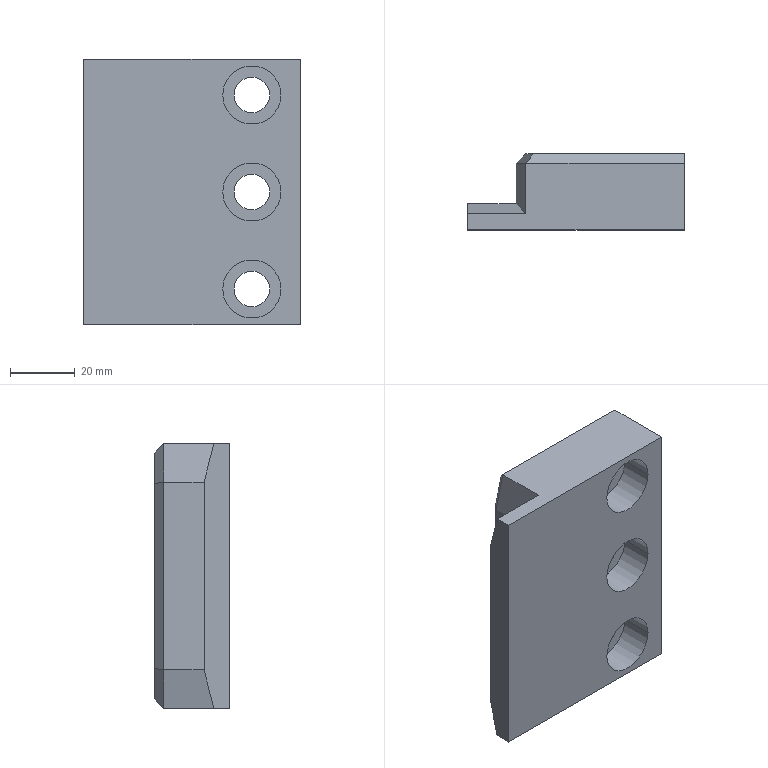Component | SolidWorks | EE8-213-_-_O-1 | 1 solid | 32 faces | box 67 x 23.5 x 82 mm | volume 96594 mm3 | plane 20 | cylinder 12 | commonest cylinder face diameters 18 x6 11 x6
build123d program:
from build123d import *
from OCP.BRepFilletAPI import BRepFilletAPI_MakeChamfer

# Parameters (mm, degrees)
EXTRUDE1_DEPTH                                       = 41
CHAMFER1_SIZE                                        = 3
CHAMFER1_SIZE2                                       = 12
CHAMFER2_SIZE                                        = 12
CHAMFER2_SIZE2                                       = 3
CHAMFER3_SIZE                                        = 3
COUNTERBORE_FOR_M10_SOCKET_HEAD_CAP_SCRE_D           = 11
COUNTERBORE_FOR_M10_SOCKET_HEAD_CAP_SCRE_CBORE_D     = 18
COUNTERBORE_FOR_M10_SOCKET_HEAD_CAP_SCRE_CBORE_DEPTH = 10


with BuildPart() as part:
    # Sketch1 → Extrude1 (new, symmetric)
    with BuildSketch(Plane(origin=(0, 0, 0), x_dir=(0, 0, -1), z_dir=(1, 0, 0))):
        Polygon((0, 0), (0, 23.5), (-52, 23.5), (-52, 8), (-67, 8), (-67, 0), align=None)
    extrude(amount=EXTRUDE1_DEPTH, both=True)

    # Chamfer1
    chamfer1_edges = [part.edges().sort_by_distance(p)[0] for p in [
        (-41, 8, 59.5),
        (-41, 15.75, 52),
    ]]
    chamfer1_side = [part.faces().sort_by_distance(p)[0] for p in [
        (-41, 11.057, 28.996),
    ]]
    chamfer(chamfer1_edges, length=CHAMFER1_SIZE, length2=CHAMFER1_SIZE2, reference=chamfer1_side[0])

    # Chamfer2: one chamfer whose edges measure the first distance from different faces: ONE call of the kernel's chamfer builder (chamfer() names one face for all edges)
    chamfer2_edges_1 = [part.edges().sort_by_distance(p)[0] for p in [
        (41, 15.75, 52),
    ]]
    chamfer2_side_1 = [part.faces().sort_by_distance(p)[0] for p in [
        (6, 15.75, 52),
    ]]
    chamfer2_edges_2 = [part.edges().sort_by_distance(p)[0] for p in [
        (41, 8, 59.5),
    ]]
    chamfer2_side_2 = [part.faces().sort_by_distance(p)[0] for p in [
        (6, 8, 59.5),
    ]]
    chamfer2 = BRepFilletAPI_MakeChamfer(part.part.solid().wrapped)
    for e in chamfer2_edges_1:
        chamfer2.Add(CHAMFER2_SIZE, CHAMFER2_SIZE2, e.wrapped, chamfer2_side_1[0].wrapped)  # the first distance lies on this face
    for e in chamfer2_edges_2:
        chamfer2.Add(CHAMFER2_SIZE, CHAMFER2_SIZE2, e.wrapped, chamfer2_side_2[0].wrapped)  # the first distance lies on this face
    add(Compound.cast(chamfer2.Shape()), mode=Mode.REPLACE)

    # Chamfer3
    chamfer3_edges = [part.edges().sort_by_distance(p)[0] for p in [
        (41, 23.5, 24.5),
        (-35, 23.5, 50.5),
        (0, 23.5, 52),
        (35, 23.5, 50.5),
        (-41, 23.5, 24.5),
    ]]
    chamfer(chamfer3_edges, length=CHAMFER3_SIZE)

    # Counterbore for M10 Socket Head Cap Scre (through all)
    with Locations(Plane.XZ):
        with Locations((0, 15), (-30, 15), (30, 15)):
            CounterBoreHole(COUNTERBORE_FOR_M10_SOCKET_HEAD_CAP_SCRE_D / 2, COUNTERBORE_FOR_M10_SOCKET_HEAD_CAP_SCRE_CBORE_D / 2, COUNTERBORE_FOR_M10_SOCKET_HEAD_CAP_SCRE_CBORE_DEPTH)


solid = part.part

# Placed as in the assembly
solid = solid.moved(Location((15, -23.5, 245), (0, -90, 0)))
STEP:
#1=CARTESIAN_POINT('',(-0.3543,-0.5315,8.465));
#2=VERTEX_POINT('',#1);
#3=CARTESIAN_POINT('',(0.3543,-0.5315,8.465));
#4=VERTEX_POINT('',#3);
#5=CARTESIAN_POINT('',(0.,-0.5315,8.465));
#6=DIRECTION('',(0.,-1.,0.));
#7=DIRECTION('',(1.,0.,-0.));
#8=AXIS2_PLACEMENT_3D('',#5,#6,#7);
#9=CIRCLE('',#8,0.3543);
#10=EDGE_CURVE('',#2,#4,#9,.T.);
#11=ORIENTED_EDGE('',*,*,#10,.F.);
#12=CARTESIAN_POINT('',(-0.3543,-0.9252,8.465));
#13=VERTEX_POINT('',#12);
#14=CARTESIAN_POINT('',(-0.3543,-0.9252,8.465));
#15=DIRECTION('',(0.,-1.,0.));
#16=VECTOR('',#15,39.37);
#17=LINE('',#14,#16);
#18=EDGE_CURVE('',#2,#13,#17,.T.);
#19=ORIENTED_EDGE('',*,*,#18,.T.);
#20=CARTESIAN_POINT('',(0.3543,-0.9252,8.465));
#21=VERTEX_POINT('',#20);
#22=CARTESIAN_POINT('',(0.,-0.9252,8.465));
#23=DIRECTION('',(0.,-1.,0.));
#24=DIRECTION('',(1.,0.,-0.));
#25=AXIS2_PLACEMENT_3D('',#22,#23,#24);
#26=CIRCLE('',#25,0.3543);
#27=EDGE_CURVE('',#13,#21,#26,.T.);
#28=ORIENTED_EDGE('',*,*,#27,.T.);
#29=CARTESIAN_POINT('',(0.3543,-0.9252,8.465));
#30=DIRECTION('',(0.,-1.,0.));
#31=VECTOR('',#30,39.37);
#32=LINE('',#29,#31);
#33=EDGE_CURVE('',#4,#21,#32,.T.);
#34=ORIENTED_EDGE('',*,*,#33,.F.);
#35=EDGE_LOOP('',(#11,#19,#28,#34));
#36=FACE_OUTER_BOUND('',#35,.T.);
#37=CARTESIAN_POINT('',(0.,-0.9252,8.465));
#38=DIRECTION('',(0.,-1.,0.));
#39=DIRECTION('',(1.,0.,-0.));
#40=AXIS2_PLACEMENT_3D('',#37,#38,#39);
#41=CYLINDRICAL_SURFACE('',#40,0.3543);
#42=ADVANCED_FACE('',(#36),#41,.F.);
#43=CARTESIAN_POINT('',(-0.2165,0.,8.465));
#44=VERTEX_POINT('',#43);
#45=CARTESIAN_POINT('',(0.2165,0.,8.465));
#46=VERTEX_POINT('',#45);
#47=CARTESIAN_POINT('',(0.,0.,8.465));
#48=DIRECTION('',(0.,-1.,0.));
#49=DIRECTION('',(1.,0.,-0.));
#50=AXIS2_PLACEMENT_3D('',#47,#48,#49);
#51=CIRCLE('',#50,0.2165);
#52=EDGE_CURVE('',#44,#46,#51,.T.);
#53=ORIENTED_EDGE('',*,*,#52,.F.);
#54=CARTESIAN_POINT('',(-0.2165,-0.5315,8.465));
#55=VERTEX_POINT('',#54);
#56=CARTESIAN_POINT('',(-0.2165,-0.9252,8.465));
#57=DIRECTION('',(0.,-1.,0.));
#58=VECTOR('',#57,39.37);
#59=LINE('',#56,#58);
#60=EDGE_CURVE('',#44,#55,#59,.T.);
#61=ORIENTED_EDGE('',*,*,#60,.T.);
#62=CARTESIAN_POINT('',(0.2165,-0.5315,8.465));
#63=VERTEX_POINT('',#62);
#64=CARTESIAN_POINT('',(0.,-0.5315,8.465));
#65=DIRECTION('',(0.,-1.,0.));
#66=DIRECTION('',(1.,0.,-0.));
#67=AXIS2_PLACEMENT_3D('',#64,#65,#66);
#68=CIRCLE('',#67,0.2165);
#69=EDGE_CURVE('',#55,#63,#68,.T.);
#70=ORIENTED_EDGE('',*,*,#69,.T.);
#71=CARTESIAN_POINT('',(0.2165,-0.9252,8.465));
#72=DIRECTION('',(0.,-1.,0.));
#73=VECTOR('',#72,39.37);
#74=LINE('',#71,#73);
#75=EDGE_CURVE('',#46,#63,#74,.T.);
#76=ORIENTED_EDGE('',*,*,#75,.F.);
#77=EDGE_LOOP('',(#53,#61,#70,#76));
#78=FACE_OUTER_BOUND('',#77,.T.);
#79=CARTESIAN_POINT('',(0.,-0.9252,8.465));
#80=DIRECTION('',(0.,-1.,0.));
#81=DIRECTION('',(1.,0.,-0.));
#82=AXIS2_PLACEMENT_3D('',#79,#80,#81);
#83=CYLINDRICAL_SURFACE('',#82,0.2165);
#84=ADVANCED_FACE('',(#78),#83,.F.);
#85=CARTESIAN_POINT('',(-0.3543,-0.5315,10.827));
#86=VERTEX_POINT('',#85);
#87=CARTESIAN_POINT('',(0.3543,-0.5315,10.827));
#88=VERTEX_POINT('',#87);
#89=CARTESIAN_POINT('',(0.,-0.5315,10.827));
#90=DIRECTION('',(0.,-1.,0.));
#91=DIRECTION('',(1.,0.,-0.));
#92=AXIS2_PLACEMENT_3D('',#89,#90,#91);
#93=CIRCLE('',#92,0.3543);
#94=EDGE_CURVE('',#86,#88,#93,.T.);
#95=ORIENTED_EDGE('',*,*,#94,.F.);
#96=CARTESIAN_POINT('',(-0.3543,-0.9252,10.827));
#97=VERTEX_POINT('',#96);
#98=CARTESIAN_POINT('',(-0.3543,-0.9252,10.827));
#99=DIRECTION('',(0.,-1.,0.));
#100=VECTOR('',#99,39.37);
#101=LINE('',#98,#100);
#102=EDGE_CURVE('',#86,#97,#101,.T.);
#103=ORIENTED_EDGE('',*,*,#102,.T.);
#104=CARTESIAN_POINT('',(0.3543,-0.9252,10.827));
#105=VERTEX_POINT('',#104);
#106=CARTESIAN_POINT('',(0.,-0.9252,10.827));
#107=DIRECTION('',(0.,-1.,0.));
#108=DIRECTION('',(1.,0.,-0.));
#109=AXIS2_PLACEMENT_3D('',#106,#107,#108);
#110=CIRCLE('',#109,0.3543);
#111=EDGE_CURVE('',#97,#105,#110,.T.);
#112=ORIENTED_EDGE('',*,*,#111,.T.);
#113=CARTESIAN_POINT('',(0.3543,-0.9252,10.827));
#114=DIRECTION('',(0.,-1.,0.));
#115=VECTOR('',#114,39.37);
#116=LINE('',#113,#115);
#117=EDGE_CURVE('',#88,#105,#116,.T.);
#118=ORIENTED_EDGE('',*,*,#117,.F.);
#119=EDGE_LOOP('',(#95,#103,#112,#118));
#120=FACE_OUTER_BOUND('',#119,.T.);
#121=CARTESIAN_POINT('',(0.,-0.9252,10.827));
#122=DIRECTION('',(0.,-1.,0.));
#123=DIRECTION('',(1.,0.,-0.));
#124=AXIS2_PLACEMENT_3D('',#121,#122,#123);
#125=CYLINDRICAL_SURFACE('',#124,0.3543);
#126=ADVANCED_FACE('',(#120),#125,.F.);
#127=CARTESIAN_POINT('',(-0.2165,0.,10.827));
#128=VERTEX_POINT('',#127);
#129=CARTESIAN_POINT('',(0.2165,0.,10.827));
#130=VERTEX_POINT('',#129);
#131=CARTESIAN_POINT('',(0.,0.,10.827));
#132=DIRECTION('',(0.,-1.,0.));
#133=DIRECTION('',(1.,0.,0.));
#134=AXIS2_PLACEMENT_3D('',#131,#132,#133);
#135=CIRCLE('',#134,0.2165);
#136=EDGE_CURVE('',#128,#130,#135,.T.);
#137=ORIENTED_EDGE('',*,*,#136,.F.);
#138=CARTESIAN_POINT('',(-0.2165,-0.5315,10.827));
#139=VERTEX_POINT('',#138);
#140=CARTESIAN_POINT('',(-0.2165,-0.9252,10.827));
#141=DIRECTION('',(0.,-1.,0.));
#142=VECTOR('',#141,39.37);
#143=LINE('',#140,#142);
#144=EDGE_CURVE('',#128,#139,#143,.T.);
#145=ORIENTED_EDGE('',*,*,#144,.T.);
#146=CARTESIAN_POINT('',(0.2165,-0.5315,10.827));
#147=VERTEX_POINT('',#146);
#148=CARTESIAN_POINT('',(0.,-0.5315,10.827));
#149=DIRECTION('',(0.,-1.,0.));
#150=DIRECTION('',(1.,0.,0.));
#151=AXIS2_PLACEMENT_3D('',#148,#149,#150);
#152=CIRCLE('',#151,0.2165);
#153=EDGE_CURVE('',#139,#147,#152,.T.);
#154=ORIENTED_EDGE('',*,*,#153,.T.);
#155=CARTESIAN_POINT('',(0.2165,-0.9252,10.827));
#156=DIRECTION('',(0.,-1.,0.));
#157=VECTOR('',#156,39.37);
#158=LINE('',#155,#157);
#159=EDGE_CURVE('',#130,#147,#158,.T.);
#160=ORIENTED_EDGE('',*,*,#159,.F.);
#161=EDGE_LOOP('',(#137,#145,#154,#160));
#162=FACE_OUTER_BOUND('',#161,.T.);
#163=CARTESIAN_POINT('',(0.,-0.9252,10.827));
#164=DIRECTION('',(0.,-1.,0.));
#165=DIRECTION('',(1.,0.,0.));
#166=AXIS2_PLACEMENT_3D('',#163,#164,#165);
#167=CYLINDRICAL_SURFACE('',#166,0.2165);
#168=ADVANCED_FACE('',(#162),#167,.F.);
#169=CARTESIAN_POINT('',(-0.3543,-0.5315,9.646));
#170=VERTEX_POINT('',#169);
#171=CARTESIAN_POINT('',(0.3543,-0.5315,9.646));
#172=VERTEX_POINT('',#171);
#173=CARTESIAN_POINT('',(0.,-0.5315,9.646));
#174=DIRECTION('',(0.,-1.,0.));
#175=DIRECTION('',(1.,0.,-0.));
#176=AXIS2_PLACEMENT_3D('',#173,#174,#175);
#177=CIRCLE('',#176,0.3543);
#178=EDGE_CURVE('',#170,#172,#177,.T.);
#179=ORIENTED_EDGE('',*,*,#178,.F.);
#180=CARTESIAN_POINT('',(-0.3543,-0.9252,9.646));
#181=VERTEX_POINT('',#180);
#182=CARTESIAN_POINT('',(-0.3543,-0.9252,9.646));
#183=DIRECTION('',(0.,-1.,0.));
#184=VECTOR('',#183,39.37);
#185=LINE('',#182,#184);
#186=EDGE_CURVE('',#170,#181,#185,.T.);
#187=ORIENTED_EDGE('',*,*,#186,.T.);
#188=CARTESIAN_POINT('',(0.3543,-0.9252,9.646));
#189=VERTEX_POINT('',#188);
#190=CARTESIAN_POINT('',(0.,-0.9252,9.646));
#191=DIRECTION('',(0.,-1.,0.));
#192=DIRECTION('',(1.,0.,-0.));
#193=AXIS2_PLACEMENT_3D('',#190,#191,#192);
#194=CIRCLE('',#193,0.3543);
#195=EDGE_CURVE('',#181,#189,#194,.T.);
#196=ORIENTED_EDGE('',*,*,#195,.T.);
#197=CARTESIAN_POINT('',(0.3543,-0.9252,9.646));
#198=DIRECTION('',(0.,-1.,0.));
#199=VECTOR('',#198,39.37);
#200=LINE('',#197,#199);
#201=EDGE_CURVE('',#172,#189,#200,.T.);
#202=ORIENTED_EDGE('',*,*,#201,.F.);
#203=EDGE_LOOP('',(#179,#187,#196,#202));
#204=FACE_OUTER_BOUND('',#203,.T.);
#205=CARTESIAN_POINT('',(0.,-0.9252,9.646));
#206=DIRECTION('',(0.,-1.,0.));
#207=DIRECTION('',(1.,0.,-0.));
#208=AXIS2_PLACEMENT_3D('',#205,#206,#207);
#209=CYLINDRICAL_SURFACE('',#208,0.3543);
#210=ADVANCED_FACE('',(#204),#209,.F.);
#211=CARTESIAN_POINT('',(-0.2165,0.,9.646));
#212=VERTEX_POINT('',#211);
#213=CARTESIAN_POINT('',(0.2165,0.,9.646));
#214=VERTEX_POINT('',#213);
#215=CARTESIAN_POINT('',(0.,0.,9.646));
#216=DIRECTION('',(0.,-1.,0.));
#217=DIRECTION('',(1.,0.,-0.));
#218=AXIS2_PLACEMENT_3D('',#215,#216,#217);
#219=CIRCLE('',#218,0.2165);
#220=EDGE_CURVE('',#212,#214,#219,.T.);
#221=ORIENTED_EDGE('',*,*,#220,.F.);
#222=CARTESIAN_POINT('',(-0.2165,-0.5315,9.646));
#223=VERTEX_POINT('',#222);
#224=CARTESIAN_POINT('',(-0.2165,-0.9252,9.646));
#225=DIRECTION('',(0.,-1.,0.));
#226=VECTOR('',#225,39.37);
#227=LINE('',#224,#226);
#228=EDGE_CURVE('',#212,#223,#227,.T.);
#229=ORIENTED_EDGE('',*,*,#228,.T.);
#230=CARTESIAN_POINT('',(0.2165,-0.5315,9.646));
#231=VERTEX_POINT('',#230);
#232=CARTESIAN_POINT('',(0.,-0.5315,9.646));
#233=DIRECTION('',(0.,-1.,0.));
#234=DIRECTION('',(1.,0.,-0.));
#235=AXIS2_PLACEMENT_3D('',#232,#233,#234);
#236=CIRCLE('',#235,0.2165);
#237=EDGE_CURVE('',#223,#231,#236,.T.);
#238=ORIENTED_EDGE('',*,*,#237,.T.);
#239=CARTESIAN_POINT('',(0.2165,-0.9252,9.646));
#240=DIRECTION('',(0.,-1.,0.));
#241=VECTOR('',#240,39.37);
#242=LINE('',#239,#241);
#243=EDGE_CURVE('',#214,#231,#242,.T.);
#244=ORIENTED_EDGE('',*,*,#243,.F.);
#245=EDGE_LOOP('',(#221,#229,#238,#244));
#246=FACE_OUTER_BOUND('',#245,.T.);
#247=CARTESIAN_POINT('',(0.,-0.9252,9.646));
#248=DIRECTION('',(0.,-1.,0.));
#249=DIRECTION('',(1.,0.,-0.));
#250=AXIS2_PLACEMENT_3D('',#247,#248,#249);
#251=CYLINDRICAL_SURFACE('',#250,0.2165);
#252=ADVANCED_FACE('',(#246),#251,.F.);
#253=CARTESIAN_POINT('',(0.,-0.9252,8.465));
#254=DIRECTION('',(0.,-1.,0.));
#255=DIRECTION('',(1.,0.,-0.));
#256=AXIS2_PLACEMENT_3D('',#253,#254,#255);
#257=CIRCLE('',#256,0.3543);
#258=EDGE_CURVE('',#21,#13,#257,.T.);
#259=ORIENTED_EDGE('',*,*,#258,.F.);
#260=ORIENTED_EDGE('',*,*,#27,.F.);
#261=EDGE_LOOP('',(#259,#260));
#262=FACE_BOUND('',#261,.T.);
#263=CARTESIAN_POINT('',(0.,-0.9252,10.827));
#264=DIRECTION('',(0.,-1.,0.));
#265=DIRECTION('',(1.,0.,-0.));
#266=AXIS2_PLACEMENT_3D('',#263,#264,#265);
#267=CIRCLE('',#266,0.3543);
#268=EDGE_CURVE('',#105,#97,#267,.T.);
#269=ORIENTED_EDGE('',*,*,#268,.F.);
#270=ORIENTED_EDGE('',*,*,#111,.F.);
#271=EDGE_LOOP('',(#269,#270));
#272=FACE_BOUND('',#271,.T.);
#273=CARTESIAN_POINT('',(0.,-0.9252,9.646));
#274=DIRECTION('',(0.,-1.,0.));
#275=DIRECTION('',(1.,0.,-0.));
#276=AXIS2_PLACEMENT_3D('',#273,#274,#275);
#277=CIRCLE('',#276,0.3543);
#278=EDGE_CURVE('',#189,#181,#277,.T.);
#279=ORIENTED_EDGE('',*,*,#278,.F.);
#280=ORIENTED_EDGE('',*,*,#195,.F.);
#281=EDGE_LOOP('',(#279,#280));
#282=FACE_BOUND('',#281,.T.);
#283=CARTESIAN_POINT('',(-2.047,-0.9252,8.031));
#284=VERTEX_POINT('',#283);
#285=CARTESIAN_POINT('',(0.5906,-0.9252,8.031));
#286=VERTEX_POINT('',#285);
#287=CARTESIAN_POINT('',(-2.047,-0.9252,8.031));
#288=DIRECTION('',(1.,0.,-0.));
#289=VECTOR('',#288,39.37);
#290=LINE('',#287,#289);
#291=EDGE_CURVE('',#284,#286,#290,.T.);
#292=ORIENTED_EDGE('',*,*,#291,.T.);
#293=CARTESIAN_POINT('',(0.5906,-0.9252,11.26));
#294=VERTEX_POINT('',#293);
#295=CARTESIAN_POINT('',(0.5906,-0.9252,11.26));
#296=DIRECTION('',(-0.,0.,-1.));
#297=VECTOR('',#296,39.37);
#298=LINE('',#295,#297);
#299=EDGE_CURVE('',#294,#286,#298,.T.);
#300=ORIENTED_EDGE('',*,*,#299,.F.);
#301=CARTESIAN_POINT('',(-2.047,-0.9252,11.26));
#302=VERTEX_POINT('',#301);
#303=CARTESIAN_POINT('',(-2.047,-0.9252,11.26));
#304=DIRECTION('',(1.,0.,-0.));
#305=VECTOR('',#304,39.37);
#306=LINE('',#303,#305);
#307=EDGE_CURVE('',#302,#294,#306,.T.);
#308=ORIENTED_EDGE('',*,*,#307,.F.);
#309=CARTESIAN_POINT('',(-2.047,-0.9252,11.26));
#310=DIRECTION('',(-0.,0.,-1.));
#311=VECTOR('',#310,39.37);
#312=LINE('',#309,#311);
#313=EDGE_CURVE('',#302,#284,#312,.T.);
#314=ORIENTED_EDGE('',*,*,#313,.T.);
#315=EDGE_LOOP('',(#292,#300,#308,#314));
#316=FACE_OUTER_BOUND('',#315,.T.);
#317=CARTESIAN_POINT('',(-2.047,-0.9252,11.26));
#318=DIRECTION('',(0.,1.,0.));
#319=DIRECTION('',(-1.,0.,0.));
#320=AXIS2_PLACEMENT_3D('',#317,#318,#319);
#321=PLANE('',#320);
#322=ADVANCED_FACE('',(#262,#272,#282,#316),#321,.F.);
#323=CARTESIAN_POINT('',(0.5906,-0.1181,8.031));
#324=VERTEX_POINT('',#323);
#325=CARTESIAN_POINT('',(0.5906,-0.9252,8.031));
#326=DIRECTION('',(0.,1.,0.));
#327=VECTOR('',#326,39.37);
#328=LINE('',#325,#327);
#329=EDGE_CURVE('',#286,#324,#328,.T.);
#330=ORIENTED_EDGE('',*,*,#329,.T.);
#331=CARTESIAN_POINT('',(0.5906,0.,8.15));
#332=VERTEX_POINT('',#331);
#333=CARTESIAN_POINT('',(0.5906,0.,8.15));
#334=DIRECTION('',(0.,0.7071,0.7071));
#335=VECTOR('',#334,39.37);
#336=LINE('',#333,#335);
#337=EDGE_CURVE('',#324,#332,#336,.T.);
#338=ORIENTED_EDGE('',*,*,#337,.T.);
#339=CARTESIAN_POINT('',(0.5906,0.,11.142));
#340=VERTEX_POINT('',#339);
#341=CARTESIAN_POINT('',(0.5906,0.,11.26));
#342=DIRECTION('',(-0.,0.,-1.));
#343=VECTOR('',#342,39.37);
#344=LINE('',#341,#343);
#345=EDGE_CURVE('',#340,#332,#344,.T.);
#346=ORIENTED_EDGE('',*,*,#345,.F.);
#347=CARTESIAN_POINT('',(0.5906,-0.1181,11.26));
#348=VERTEX_POINT('',#347);
#349=CARTESIAN_POINT('',(0.5906,-0.1181,11.26));
#350=DIRECTION('',(0.,-0.7071,0.7071));
#351=VECTOR('',#350,39.37);
#352=LINE('',#349,#351);
#353=EDGE_CURVE('',#340,#348,#352,.T.);
#354=ORIENTED_EDGE('',*,*,#353,.T.);
#355=CARTESIAN_POINT('',(0.5906,-0.9252,11.26));
#356=DIRECTION('',(0.,1.,0.));
#357=VECTOR('',#356,39.37);
#358=LINE('',#355,#357);
#359=EDGE_CURVE('',#294,#348,#358,.T.);
#360=ORIENTED_EDGE('',*,*,#359,.F.);
#361=ORIENTED_EDGE('',*,*,#299,.T.);
#362=EDGE_LOOP('',(#330,#338,#346,#354,#360,#361));
#363=FACE_OUTER_BOUND('',#362,.T.);
#364=CARTESIAN_POINT('',(0.5906,-0.9252,11.26));
#365=DIRECTION('',(-1.,0.,0.));
#366=DIRECTION('',(0.,0.,1.));
#367=AXIS2_PLACEMENT_3D('',#364,#365,#366);
#368=PLANE('',#367);
#369=ADVANCED_FACE('',(#363),#368,.F.);
#370=CARTESIAN_POINT('',(0.,0.,8.465));
#371=DIRECTION('',(0.,-1.,0.));
#372=DIRECTION('',(1.,0.,-0.));
#373=AXIS2_PLACEMENT_3D('',#370,#371,#372);
#374=CIRCLE('',#373,0.2165);
#375=EDGE_CURVE('',#46,#44,#374,.T.);
#376=ORIENTED_EDGE('',*,*,#375,.T.);
#377=ORIENTED_EDGE('',*,*,#52,.T.);
#378=EDGE_LOOP('',(#376,#377));
#379=FACE_BOUND('',#378,.T.);
#380=CARTESIAN_POINT('',(0.,0.,10.827));
#381=DIRECTION('',(0.,-1.,0.));
#382=DIRECTION('',(1.,0.,0.));
#383=AXIS2_PLACEMENT_3D('',#380,#381,#382);
#384=CIRCLE('',#383,0.2165);
#385=EDGE_CURVE('',#130,#128,#384,.T.);
#386=ORIENTED_EDGE('',*,*,#385,.T.);
#387=ORIENTED_EDGE('',*,*,#136,.T.);
#388=EDGE_LOOP('',(#386,#387));
#389=FACE_BOUND('',#388,.T.);
#390=CARTESIAN_POINT('',(0.,0.,9.646));
#391=DIRECTION('',(0.,-1.,0.));
#392=DIRECTION('',(1.,0.,-0.));
#393=AXIS2_PLACEMENT_3D('',#390,#391,#392);
#394=CIRCLE('',#393,0.2165);
#395=EDGE_CURVE('',#214,#212,#394,.T.);
#396=ORIENTED_EDGE('',*,*,#395,.T.);
#397=ORIENTED_EDGE('',*,*,#220,.T.);
#398=EDGE_LOOP('',(#396,#397));
#399=FACE_BOUND('',#398,.T.);
#400=ORIENTED_EDGE('',*,*,#345,.T.);
#401=CARTESIAN_POINT('',(-1.246,0.,8.15));
#402=VERTEX_POINT('',#401);
#403=CARTESIAN_POINT('',(0.5906,0.,8.15));
#404=DIRECTION('',(-1.,-0.,0.));
#405=VECTOR('',#404,39.37);
#406=LINE('',#403,#405);
#407=EDGE_CURVE('',#332,#402,#406,.T.);
#408=ORIENTED_EDGE('',*,*,#407,.T.);
#409=CARTESIAN_POINT('',(-1.339,0.,8.518));
#410=VERTEX_POINT('',#409);
#411=CARTESIAN_POINT('',(-1.342,0.,8.533));
#412=DIRECTION('',(-0.2425,-0.,0.9701));
#413=VECTOR('',#412,39.37);
#414=LINE('',#411,#413);
#415=EDGE_CURVE('',#402,#410,#414,.T.);
#416=ORIENTED_EDGE('',*,*,#415,.T.);
#417=CARTESIAN_POINT('',(-1.339,0.,10.773));
#418=VERTEX_POINT('',#417);
#419=CARTESIAN_POINT('',(-1.339,0.,11.26));
#420=DIRECTION('',(0.,0.,1.));
#421=VECTOR('',#420,39.37);
#422=LINE('',#419,#421);
#423=EDGE_CURVE('',#410,#418,#422,.T.);
#424=ORIENTED_EDGE('',*,*,#423,.T.);
#425=CARTESIAN_POINT('',(-1.246,0.,11.142));
#426=VERTEX_POINT('',#425);
#427=CARTESIAN_POINT('',(-1.224,0.,11.231));
#428=DIRECTION('',(0.2425,0.,0.9701));
#429=VECTOR('',#428,39.37);
#430=LINE('',#427,#429);
#431=EDGE_CURVE('',#418,#426,#430,.T.);
#432=ORIENTED_EDGE('',*,*,#431,.T.);
#433=CARTESIAN_POINT('',(0.5906,0.,11.142));
#434=DIRECTION('',(1.,0.,-0.));
#435=VECTOR('',#434,39.37);
#436=LINE('',#433,#435);
#437=EDGE_CURVE('',#426,#340,#436,.T.);
#438=ORIENTED_EDGE('',*,*,#437,.T.);
#439=EDGE_LOOP('',(#400,#408,#416,#424,#432,#438));
#440=FACE_OUTER_BOUND('',#439,.T.);
#441=CARTESIAN_POINT('',(0.5906,0.,11.26));
#442=DIRECTION('',(0.,-1.,-0.));
#443=DIRECTION('',(1.,0.,-0.));
#444=AXIS2_PLACEMENT_3D('',#441,#442,#443);
#445=PLANE('',#444);
#446=ADVANCED_FACE('',(#379,#389,#399,#440),#445,.F.);
#447=CARTESIAN_POINT('',(-1.457,-0.6102,10.787));
#448=VERTEX_POINT('',#447);
#449=CARTESIAN_POINT('',(-1.457,-0.1181,10.787));
#450=VERTEX_POINT('',#449);
#451=CARTESIAN_POINT('',(-1.457,0.,10.787));
#452=DIRECTION('',(-0.,1.,0.));
#453=VECTOR('',#452,39.37);
#454=LINE('',#451,#453);
#455=EDGE_CURVE('',#448,#450,#454,.T.);
#456=ORIENTED_EDGE('',*,*,#455,.T.);
#457=CARTESIAN_POINT('',(-1.457,-0.1181,8.504));
#458=VERTEX_POINT('',#457);
#459=CARTESIAN_POINT('',(-1.457,-0.1181,11.26));
#460=DIRECTION('',(-0.,0.,-1.));
#461=VECTOR('',#460,39.37);
#462=LINE('',#459,#461);
#463=EDGE_CURVE('',#450,#458,#462,.T.);
#464=ORIENTED_EDGE('',*,*,#463,.T.);
#465=CARTESIAN_POINT('',(-1.457,-0.6102,8.504));
#466=VERTEX_POINT('',#465);
#467=CARTESIAN_POINT('',(-1.457,0.,8.504));
#468=DIRECTION('',(0.,-1.,-0.));
#469=VECTOR('',#468,39.37);
#470=LINE('',#467,#469);
#471=EDGE_CURVE('',#458,#466,#470,.T.);
#472=ORIENTED_EDGE('',*,*,#471,.T.);
#473=CARTESIAN_POINT('',(-1.457,-0.6102,11.26));
#474=DIRECTION('',(-0.,0.,-1.));
#475=VECTOR('',#474,39.37);
#476=LINE('',#473,#475);
#477=EDGE_CURVE('',#448,#466,#476,.T.);
#478=ORIENTED_EDGE('',*,*,#477,.F.);
#479=EDGE_LOOP('',(#456,#464,#472,#478));
#480=FACE_OUTER_BOUND('',#479,.T.);
#481=CARTESIAN_POINT('',(-1.457,0.,11.26));
#482=DIRECTION('',(1.,0.,-0.));
#483=DIRECTION('',(-0.,1.,0.));
#484=AXIS2_PLACEMENT_3D('',#481,#482,#483);
#485=PLANE('',#484);
#486=ADVANCED_FACE('',(#480),#485,.F.);
#487=CARTESIAN_POINT('',(-2.047,-0.6102,10.787));
#488=VERTEX_POINT('',#487);
#489=CARTESIAN_POINT('',(-2.047,-0.6102,8.504));
#490=VERTEX_POINT('',#489);
#491=CARTESIAN_POINT('',(-2.047,-0.6102,11.26));
#492=DIRECTION('',(-0.,0.,-1.));
#493=VECTOR('',#492,39.37);
#494=LINE('',#491,#493);
#495=EDGE_CURVE('',#488,#490,#494,.T.);
#496=ORIENTED_EDGE('',*,*,#495,.F.);
#497=CARTESIAN_POINT('',(-1.457,-0.6102,10.787));
#498=DIRECTION('',(1.,0.,-0.));
#499=VECTOR('',#498,39.37);
#500=LINE('',#497,#499);
#501=EDGE_CURVE('',#488,#448,#500,.T.);
#502=ORIENTED_EDGE('',*,*,#501,.T.);
#503=ORIENTED_EDGE('',*,*,#477,.T.);
#504=CARTESIAN_POINT('',(-1.457,-0.6102,8.504));
#505=DIRECTION('',(-1.,-0.,0.));
#506=VECTOR('',#505,39.37);
#507=LINE('',#504,#506);
#508=EDGE_CURVE('',#466,#490,#507,.T.);
#509=ORIENTED_EDGE('',*,*,#508,.T.);
#510=EDGE_LOOP('',(#496,#502,#503,#509));
#511=FACE_OUTER_BOUND('',#510,.T.);
#512=CARTESIAN_POINT('',(-1.457,-0.6102,11.26));
#513=DIRECTION('',(0.,-1.,-0.));
#514=DIRECTION('',(1.,0.,-0.));
#515=AXIS2_PLACEMENT_3D('',#512,#513,#514);
#516=PLANE('',#515);
#517=ADVANCED_FACE('',(#511),#516,.F.);
#518=CARTESIAN_POINT('',(-2.047,-0.7283,11.26));
#519=VERTEX_POINT('',#518);
#520=CARTESIAN_POINT('',(-2.047,-0.6102,11.26));
#521=DIRECTION('',(0.,-1.,0.));
#522=VECTOR('',#521,39.37);
#523=LINE('',#520,#522);
#524=EDGE_CURVE('',#519,#302,#523,.T.);
#525=ORIENTED_EDGE('',*,*,#524,.F.);
#526=CARTESIAN_POINT('',(-2.047,-0.7283,11.26));
#527=DIRECTION('',(-0.,0.2425,-0.9701));
#528=VECTOR('',#527,39.37);
#529=LINE('',#526,#528);
#530=EDGE_CURVE('',#519,#488,#529,.T.);
#531=ORIENTED_EDGE('',*,*,#530,.T.);
#532=ORIENTED_EDGE('',*,*,#495,.T.);
#533=CARTESIAN_POINT('',(-2.047,-0.7283,8.031));
#534=VERTEX_POINT('',#533);
#535=CARTESIAN_POINT('',(-2.047,-0.6102,8.504));
#536=DIRECTION('',(-0.,-0.2425,-0.9701));
#537=VECTOR('',#536,39.37);
#538=LINE('',#535,#537);
#539=EDGE_CURVE('',#490,#534,#538,.T.);
#540=ORIENTED_EDGE('',*,*,#539,.T.);
#541=CARTESIAN_POINT('',(-2.047,-0.6102,8.031));
#542=DIRECTION('',(0.,-1.,0.));
#543=VECTOR('',#542,39.37);
#544=LINE('',#541,#543);
#545=EDGE_CURVE('',#534,#284,#544,.T.);
#546=ORIENTED_EDGE('',*,*,#545,.T.);
#547=ORIENTED_EDGE('',*,*,#313,.F.);
#548=EDGE_LOOP('',(#525,#531,#532,#540,#546,#547));
#549=FACE_OUTER_BOUND('',#548,.T.);
#550=CARTESIAN_POINT('',(-2.047,-0.6102,11.26));
#551=DIRECTION('',(1.,0.,-0.));
#552=DIRECTION('',(-0.,0.,-1.));
#553=AXIS2_PLACEMENT_3D('',#550,#551,#552);
#554=PLANE('',#553);
#555=ADVANCED_FACE('',(#549),#554,.F.);
#556=ORIENTED_EDGE('',*,*,#359,.T.);
#557=CARTESIAN_POINT('',(-1.339,-0.1181,11.26));
#558=VERTEX_POINT('',#557);
#559=CARTESIAN_POINT('',(-1.339,-0.1181,11.26));
#560=DIRECTION('',(-1.,-0.,0.));
#561=VECTOR('',#560,39.37);
#562=LINE('',#559,#561);
#563=EDGE_CURVE('',#348,#558,#562,.T.);
#564=ORIENTED_EDGE('',*,*,#563,.T.);
#565=CARTESIAN_POINT('',(-1.339,-0.7283,11.26));
#566=VERTEX_POINT('',#565);
#567=CARTESIAN_POINT('',(-1.339,-0.6102,11.26));
#568=DIRECTION('',(0.,-1.,-0.));
#569=VECTOR('',#568,39.37);
#570=LINE('',#567,#569);
#571=EDGE_CURVE('',#558,#566,#570,.T.);
#572=ORIENTED_EDGE('',*,*,#571,.T.);
#573=CARTESIAN_POINT('',(-2.047,-0.7283,11.26));
#574=DIRECTION('',(-1.,-0.,0.));
#575=VECTOR('',#574,39.37);
#576=LINE('',#573,#575);
#577=EDGE_CURVE('',#566,#519,#576,.T.);
#578=ORIENTED_EDGE('',*,*,#577,.T.);
#579=ORIENTED_EDGE('',*,*,#524,.T.);
#580=ORIENTED_EDGE('',*,*,#307,.T.);
#581=EDGE_LOOP('',(#556,#564,#572,#578,#579,#580));
#582=FACE_OUTER_BOUND('',#581,.T.);
#583=CARTESIAN_POINT('',(0.5906,-0.9252,11.26));
#584=DIRECTION('',(0.,0.,1.));
#585=DIRECTION('',(1.,0.,-0.));
#586=AXIS2_PLACEMENT_3D('',#583,#584,#585);
#587=PLANE('',#586);
#588=ADVANCED_FACE('',(#582),#587,.T.);
#589=CARTESIAN_POINT('',(-1.339,-0.7283,8.031));
#590=VERTEX_POINT('',#589);
#591=CARTESIAN_POINT('',(-1.339,-0.1181,8.031));
#592=VERTEX_POINT('',#591);
#593=CARTESIAN_POINT('',(-1.339,-0.9252,8.031));
#594=DIRECTION('',(-0.,1.,0.));
#595=VECTOR('',#594,39.37);
#596=LINE('',#593,#595);
#597=EDGE_CURVE('',#590,#592,#596,.T.);
#598=ORIENTED_EDGE('',*,*,#597,.T.);
#599=CARTESIAN_POINT('',(0.5906,-0.1181,8.031));
#600=DIRECTION('',(1.,0.,-0.));
#601=VECTOR('',#600,39.37);
#602=LINE('',#599,#601);
#603=EDGE_CURVE('',#592,#324,#602,.T.);
#604=ORIENTED_EDGE('',*,*,#603,.T.);
#605=ORIENTED_EDGE('',*,*,#329,.F.);
#606=ORIENTED_EDGE('',*,*,#291,.F.);
#607=ORIENTED_EDGE('',*,*,#545,.F.);
#608=CARTESIAN_POINT('',(0.5906,-0.7283,8.031));
#609=DIRECTION('',(1.,0.,-0.));
#610=VECTOR('',#609,39.37);
#611=LINE('',#608,#610);
#612=EDGE_CURVE('',#534,#590,#611,.T.);
#613=ORIENTED_EDGE('',*,*,#612,.T.);
#614=EDGE_LOOP('',(#598,#604,#605,#606,#607,#613));
#615=FACE_OUTER_BOUND('',#614,.T.);
#616=CARTESIAN_POINT('',(0.5906,-0.9252,8.031));
#617=DIRECTION('',(0.,0.,1.));
#618=DIRECTION('',(1.,0.,-0.));
#619=AXIS2_PLACEMENT_3D('',#616,#617,#618);
#620=PLANE('',#619);
#621=ADVANCED_FACE('',(#615),#620,.F.);
#622=ORIENTED_EDGE('',*,*,#539,.F.);
#623=ORIENTED_EDGE('',*,*,#508,.F.);
#624=CARTESIAN_POINT('',(-1.491,-0.5763,8.64));
#625=DIRECTION('',(-0.2357,0.2357,0.9428));
#626=VECTOR('',#625,39.37);
#627=LINE('',#624,#626);
#628=EDGE_CURVE('',#590,#466,#627,.T.);
#629=ORIENTED_EDGE('',*,*,#628,.F.);
#630=ORIENTED_EDGE('',*,*,#612,.F.);
#631=EDGE_LOOP('',(#622,#623,#629,#630));
#632=FACE_OUTER_BOUND('',#631,.T.);
#633=CARTESIAN_POINT('',(-1.457,-0.6102,8.504));
#634=DIRECTION('',(0.,-0.9701,0.2425));
#635=DIRECTION('',(0.,0.2425,0.9701));
#636=AXIS2_PLACEMENT_3D('',#633,#634,#635);
#637=PLANE('',#636);
#638=ADVANCED_FACE('',(#632),#637,.F.);
#639=ORIENTED_EDGE('',*,*,#471,.F.);
#640=CARTESIAN_POINT('',(-1.339,-0.1181,8.031));
#641=DIRECTION('',(0.2425,0.,-0.9701));
#642=VECTOR('',#641,39.37);
#643=LINE('',#640,#642);
#644=EDGE_CURVE('',#458,#592,#643,.T.);
#645=ORIENTED_EDGE('',*,*,#644,.T.);
#646=ORIENTED_EDGE('',*,*,#597,.F.);
#647=ORIENTED_EDGE('',*,*,#628,.T.);
#648=EDGE_LOOP('',(#639,#645,#646,#647));
#649=FACE_OUTER_BOUND('',#648,.T.);
#650=CARTESIAN_POINT('',(-1.457,0.,8.504));
#651=DIRECTION('',(0.9701,0.,0.2425));
#652=DIRECTION('',(0.2425,0.,-0.9701));
#653=AXIS2_PLACEMENT_3D('',#650,#651,#652);
#654=PLANE('',#653);
#655=ADVANCED_FACE('',(#649),#654,.F.);
#656=ORIENTED_EDGE('',*,*,#530,.F.);
#657=ORIENTED_EDGE('',*,*,#577,.F.);
#658=CARTESIAN_POINT('',(-1.328,-0.7393,11.304));
#659=DIRECTION('',(0.2357,-0.2357,0.9428));
#660=VECTOR('',#659,39.37);
#661=LINE('',#658,#660);
#662=EDGE_CURVE('',#448,#566,#661,.T.);
#663=ORIENTED_EDGE('',*,*,#662,.F.);
#664=ORIENTED_EDGE('',*,*,#501,.F.);
#665=EDGE_LOOP('',(#656,#657,#663,#664));
#666=FACE_OUTER_BOUND('',#665,.T.);
#667=CARTESIAN_POINT('',(0.5906,-0.7283,11.26));
#668=DIRECTION('',(0.,0.9701,0.2425));
#669=DIRECTION('',(-0.,0.2425,-0.9701));
#670=AXIS2_PLACEMENT_3D('',#667,#668,#669);
#671=PLANE('',#670);
#672=ADVANCED_FACE('',(#666),#671,.T.);
#673=ORIENTED_EDGE('',*,*,#571,.F.);
#674=CARTESIAN_POINT('',(-1.457,-0.1181,10.787));
#675=DIRECTION('',(-0.2425,-0.,-0.9701));
#676=VECTOR('',#675,39.37);
#677=LINE('',#674,#676);
#678=EDGE_CURVE('',#558,#450,#677,.T.);
#679=ORIENTED_EDGE('',*,*,#678,.T.);
#680=ORIENTED_EDGE('',*,*,#455,.F.);
#681=ORIENTED_EDGE('',*,*,#662,.T.);
#682=EDGE_LOOP('',(#673,#679,#680,#681));
#683=FACE_OUTER_BOUND('',#682,.T.);
#684=CARTESIAN_POINT('',(-1.339,-0.9252,11.26));
#685=DIRECTION('',(-0.9701,-0.,0.2425));
#686=DIRECTION('',(0.2425,0.,0.9701));
#687=AXIS2_PLACEMENT_3D('',#684,#685,#686);
#688=PLANE('',#687);
#689=ADVANCED_FACE('',(#683),#688,.T.);
#690=ORIENTED_EDGE('',*,*,#353,.F.);
#691=ORIENTED_EDGE('',*,*,#437,.F.);
#692=CARTESIAN_POINT('',(-1.377,-0.1676,11.309));
#693=DIRECTION('',(0.4833,0.619,-0.619));
#694=VECTOR('',#693,39.37);
#695=LINE('',#692,#694);
#696=EDGE_CURVE('',#558,#426,#695,.T.);
#697=ORIENTED_EDGE('',*,*,#696,.F.);
#698=ORIENTED_EDGE('',*,*,#563,.F.);
#699=EDGE_LOOP('',(#690,#691,#697,#698));
#700=FACE_OUTER_BOUND('',#699,.T.);
#701=CARTESIAN_POINT('',(0.5906,-0.1181,11.26));
#702=DIRECTION('',(0.,0.7071,0.7071));
#703=DIRECTION('',(-0.,0.7071,-0.7071));
#704=AXIS2_PLACEMENT_3D('',#701,#702,#703);
#705=PLANE('',#704);
#706=ADVANCED_FACE('',(#700),#705,.T.);
#707=ORIENTED_EDGE('',*,*,#696,.T.);
#708=ORIENTED_EDGE('',*,*,#431,.F.);
#709=CARTESIAN_POINT('',(-1.486,-0.147,10.791));
#710=DIRECTION('',(0.7044,0.7044,-0.08672));
#711=VECTOR('',#710,39.37);
#712=LINE('',#709,#711);
#713=EDGE_CURVE('',#450,#418,#712,.T.);
#714=ORIENTED_EDGE('',*,*,#713,.F.);
#715=ORIENTED_EDGE('',*,*,#678,.F.);
#716=EDGE_LOOP('',(#707,#708,#714,#715));
#717=FACE_OUTER_BOUND('',#716,.T.);
#718=CARTESIAN_POINT('',(-1.111,0.,11.685));
#719=DIRECTION('',(-0.686,0.7071,0.1715));
#720=DIRECTION('',(-0.7177,-0.6963,0.));
#721=AXIS2_PLACEMENT_3D('',#718,#719,#720);
#722=PLANE('',#721);
#723=ADVANCED_FACE('',(#717),#722,.T.);
#724=ORIENTED_EDGE('',*,*,#713,.T.);
#725=ORIENTED_EDGE('',*,*,#423,.F.);
#726=CARTESIAN_POINT('',(-1.288,0.05025,8.525));
#727=DIRECTION('',(0.7044,0.7044,0.08672));
#728=VECTOR('',#727,39.37);
#729=LINE('',#726,#728);
#730=EDGE_CURVE('',#458,#410,#729,.T.);
#731=ORIENTED_EDGE('',*,*,#730,.F.);
#732=ORIENTED_EDGE('',*,*,#463,.F.);
#733=EDGE_LOOP('',(#724,#725,#731,#732));
#734=FACE_OUTER_BOUND('',#733,.T.);
#735=CARTESIAN_POINT('',(-1.457,-0.1181,11.26));
#736=DIRECTION('',(0.7071,-0.7071,-0.));
#737=DIRECTION('',(0.7071,0.7071,-0.));
#738=AXIS2_PLACEMENT_3D('',#735,#736,#737);
#739=PLANE('',#738);
#740=ADVANCED_FACE('',(#734),#739,.F.);
#741=ORIENTED_EDGE('',*,*,#730,.T.);
#742=ORIENTED_EDGE('',*,*,#415,.F.);
#743=CARTESIAN_POINT('',(-0.6456,0.7695,8.919));
#744=DIRECTION('',(0.4833,0.619,0.619));
#745=VECTOR('',#744,39.37);
#746=LINE('',#743,#745);
#747=EDGE_CURVE('',#592,#402,#746,.T.);
#748=ORIENTED_EDGE('',*,*,#747,.F.);
#749=ORIENTED_EDGE('',*,*,#644,.F.);
#750=EDGE_LOOP('',(#741,#742,#748,#749));
#751=FACE_OUTER_BOUND('',#750,.T.);
#752=CARTESIAN_POINT('',(-1.87,0.,10.645));
#753=DIRECTION('',(0.686,-0.7071,0.1715));
#754=DIRECTION('',(0.7177,0.6963,-0.));
#755=AXIS2_PLACEMENT_3D('',#752,#753,#754);
#756=PLANE('',#755);
#757=ADVANCED_FACE('',(#751),#756,.F.);
#758=ORIENTED_EDGE('',*,*,#337,.F.);
#759=ORIENTED_EDGE('',*,*,#603,.F.);
#760=ORIENTED_EDGE('',*,*,#747,.T.);
#761=ORIENTED_EDGE('',*,*,#407,.F.);
#762=EDGE_LOOP('',(#758,#759,#760,#761));
#763=FACE_OUTER_BOUND('',#762,.T.);
#764=CARTESIAN_POINT('',(0.5906,0.,8.15));
#765=DIRECTION('',(0.,-0.7071,0.7071));
#766=DIRECTION('',(0.,0.7071,0.7071));
#767=AXIS2_PLACEMENT_3D('',#764,#765,#766);
#768=PLANE('',#767);
#769=ADVANCED_FACE('',(#763),#768,.F.);
#770=ORIENTED_EDGE('',*,*,#228,.F.);
#771=ORIENTED_EDGE('',*,*,#395,.F.);
#772=ORIENTED_EDGE('',*,*,#243,.T.);
#773=CARTESIAN_POINT('',(0.,-0.5315,9.646));
#774=DIRECTION('',(0.,-1.,0.));
#775=DIRECTION('',(1.,0.,-0.));
#776=AXIS2_PLACEMENT_3D('',#773,#774,#775);
#777=CIRCLE('',#776,0.2165);
#778=EDGE_CURVE('',#231,#223,#777,.T.);
#779=ORIENTED_EDGE('',*,*,#778,.T.);
#780=EDGE_LOOP('',(#770,#771,#772,#779));
#781=FACE_OUTER_BOUND('',#780,.T.);
#782=CARTESIAN_POINT('',(0.,-0.9252,9.646));
#783=DIRECTION('',(0.,-1.,0.));
#784=DIRECTION('',(1.,0.,-0.));
#785=AXIS2_PLACEMENT_3D('',#782,#783,#784);
#786=CYLINDRICAL_SURFACE('',#785,0.2165);
#787=ADVANCED_FACE('',(#781),#786,.F.);
#788=ORIENTED_EDGE('',*,*,#778,.F.);
#789=ORIENTED_EDGE('',*,*,#237,.F.);
#790=EDGE_LOOP('',(#788,#789));
#791=FACE_BOUND('',#790,.T.);
#792=CARTESIAN_POINT('',(0.,-0.5315,9.646));
#793=DIRECTION('',(0.,-1.,0.));
#794=DIRECTION('',(1.,0.,-0.));
#795=AXIS2_PLACEMENT_3D('',#792,#793,#794);
#796=CIRCLE('',#795,0.3543);
#797=EDGE_CURVE('',#172,#170,#796,.T.);
#798=ORIENTED_EDGE('',*,*,#797,.T.);
#799=ORIENTED_EDGE('',*,*,#178,.T.);
#800=EDGE_LOOP('',(#798,#799));
#801=FACE_OUTER_BOUND('',#800,.T.);
#802=CARTESIAN_POINT('',(0.,-0.5315,9.862));
#803=DIRECTION('',(0.,1.,0.));
#804=DIRECTION('',(-1.,0.,0.));
#805=AXIS2_PLACEMENT_3D('',#802,#803,#804);
#806=PLANE('',#805);
#807=ADVANCED_FACE('',(#791,#801),#806,.F.);
#808=ORIENTED_EDGE('',*,*,#186,.F.);
#809=ORIENTED_EDGE('',*,*,#797,.F.);
#810=ORIENTED_EDGE('',*,*,#201,.T.);
#811=ORIENTED_EDGE('',*,*,#278,.T.);
#812=EDGE_LOOP('',(#808,#809,#810,#811));
#813=FACE_OUTER_BOUND('',#812,.T.);
#814=CARTESIAN_POINT('',(0.,-0.9252,9.646));
#815=DIRECTION('',(0.,-1.,0.));
#816=DIRECTION('',(1.,0.,-0.));
#817=AXIS2_PLACEMENT_3D('',#814,#815,#816);
#818=CYLINDRICAL_SURFACE('',#817,0.3543);
#819=ADVANCED_FACE('',(#813),#818,.F.);
#820=ORIENTED_EDGE('',*,*,#144,.F.);
#821=ORIENTED_EDGE('',*,*,#385,.F.);
#822=ORIENTED_EDGE('',*,*,#159,.T.);
#823=CARTESIAN_POINT('',(0.,-0.5315,10.827));
#824=DIRECTION('',(0.,-1.,0.));
#825=DIRECTION('',(1.,0.,0.));
#826=AXIS2_PLACEMENT_3D('',#823,#824,#825);
#827=CIRCLE('',#826,0.2165);
#828=EDGE_CURVE('',#147,#139,#827,.T.);
#829=ORIENTED_EDGE('',*,*,#828,.T.);
#830=EDGE_LOOP('',(#820,#821,#822,#829));
#831=FACE_OUTER_BOUND('',#830,.T.);
#832=CARTESIAN_POINT('',(0.,-0.9252,10.827));
#833=DIRECTION('',(0.,-1.,0.));
#834=DIRECTION('',(1.,0.,0.));
#835=AXIS2_PLACEMENT_3D('',#832,#833,#834);
#836=CYLINDRICAL_SURFACE('',#835,0.2165);
#837=ADVANCED_FACE('',(#831),#836,.F.);
#838=ORIENTED_EDGE('',*,*,#828,.F.);
#839=ORIENTED_EDGE('',*,*,#153,.F.);
#840=EDGE_LOOP('',(#838,#839));
#841=FACE_BOUND('',#840,.T.);
#842=CARTESIAN_POINT('',(0.,-0.5315,10.827));
#843=DIRECTION('',(0.,-1.,0.));
#844=DIRECTION('',(1.,0.,-0.));
#845=AXIS2_PLACEMENT_3D('',#842,#843,#844);
#846=CIRCLE('',#845,0.3543);
#847=EDGE_CURVE('',#88,#86,#846,.T.);
#848=ORIENTED_EDGE('',*,*,#847,.T.);
#849=ORIENTED_EDGE('',*,*,#94,.T.);
#850=EDGE_LOOP('',(#848,#849));
#851=FACE_OUTER_BOUND('',#850,.T.);
#852=CARTESIAN_POINT('',(0.,-0.5315,11.043));
#853=DIRECTION('',(0.,1.,0.));
#854=DIRECTION('',(-1.,0.,0.));
#855=AXIS2_PLACEMENT_3D('',#852,#853,#854);
#856=PLANE('',#855);
#857=ADVANCED_FACE('',(#841,#851),#856,.F.);
#858=ORIENTED_EDGE('',*,*,#102,.F.);
#859=ORIENTED_EDGE('',*,*,#847,.F.);
#860=ORIENTED_EDGE('',*,*,#117,.T.);
#861=ORIENTED_EDGE('',*,*,#268,.T.);
#862=EDGE_LOOP('',(#858,#859,#860,#861));
#863=FACE_OUTER_BOUND('',#862,.T.);
#864=CARTESIAN_POINT('',(0.,-0.9252,10.827));
#865=DIRECTION('',(0.,-1.,0.));
#866=DIRECTION('',(1.,0.,-0.));
#867=AXIS2_PLACEMENT_3D('',#864,#865,#866);
#868=CYLINDRICAL_SURFACE('',#867,0.3543);
#869=ADVANCED_FACE('',(#863),#868,.F.);
#870=ORIENTED_EDGE('',*,*,#60,.F.);
#871=ORIENTED_EDGE('',*,*,#375,.F.);
#872=ORIENTED_EDGE('',*,*,#75,.T.);
#873=CARTESIAN_POINT('',(0.,-0.5315,8.465));
#874=DIRECTION('',(0.,-1.,0.));
#875=DIRECTION('',(1.,0.,-0.));
#876=AXIS2_PLACEMENT_3D('',#873,#874,#875);
#877=CIRCLE('',#876,0.2165);
#878=EDGE_CURVE('',#63,#55,#877,.T.);
#879=ORIENTED_EDGE('',*,*,#878,.T.);
#880=EDGE_LOOP('',(#870,#871,#872,#879));
#881=FACE_OUTER_BOUND('',#880,.T.);
#882=CARTESIAN_POINT('',(0.,-0.9252,8.465));
#883=DIRECTION('',(0.,-1.,0.));
#884=DIRECTION('',(1.,0.,-0.));
#885=AXIS2_PLACEMENT_3D('',#882,#883,#884);
#886=CYLINDRICAL_SURFACE('',#885,0.2165);
#887=ADVANCED_FACE('',(#881),#886,.F.);
#888=ORIENTED_EDGE('',*,*,#878,.F.);
#889=ORIENTED_EDGE('',*,*,#69,.F.);
#890=EDGE_LOOP('',(#888,#889));
#891=FACE_BOUND('',#890,.T.);
#892=CARTESIAN_POINT('',(0.,-0.5315,8.465));
#893=DIRECTION('',(0.,-1.,0.));
#894=DIRECTION('',(1.,0.,-0.));
#895=AXIS2_PLACEMENT_3D('',#892,#893,#894);
#896=CIRCLE('',#895,0.3543);
#897=EDGE_CURVE('',#4,#2,#896,.T.);
#898=ORIENTED_EDGE('',*,*,#897,.T.);
#899=ORIENTED_EDGE('',*,*,#10,.T.);
#900=EDGE_LOOP('',(#898,#899));
#901=FACE_OUTER_BOUND('',#900,.T.);
#902=CARTESIAN_POINT('',(0.,-0.5315,8.681));
#903=DIRECTION('',(0.,1.,0.));
#904=DIRECTION('',(-1.,0.,0.));
#905=AXIS2_PLACEMENT_3D('',#902,#903,#904);
#906=PLANE('',#905);
#907=ADVANCED_FACE('',(#891,#901),#906,.F.);
#908=ORIENTED_EDGE('',*,*,#18,.F.);
#909=ORIENTED_EDGE('',*,*,#897,.F.);
#910=ORIENTED_EDGE('',*,*,#33,.T.);
#911=ORIENTED_EDGE('',*,*,#258,.T.);
#912=EDGE_LOOP('',(#908,#909,#910,#911));
#913=FACE_OUTER_BOUND('',#912,.T.);
#914=CARTESIAN_POINT('',(0.,-0.9252,8.465));
#915=DIRECTION('',(0.,-1.,0.));
#916=DIRECTION('',(1.,0.,-0.));
#917=AXIS2_PLACEMENT_3D('',#914,#915,#916);
#918=CYLINDRICAL_SURFACE('',#917,0.3543);
#919=ADVANCED_FACE('',(#913),#918,.F.);
#920=CLOSED_SHELL('',(#42,#84,#126,#168,#210,#252,#322,#369,#446,#486,#517,#555,#588,#621,#638,#655,#672,#689,#706,#723,#740,#757,#769,#787,#807,#819,#837,#857,#869,#887,#907,#919));
#921=MANIFOLD_SOLID_BREP('',#920);
#922=CARTESIAN_POINT('',(0.,0.,0.));
#923=DIRECTION('',(0.,0.,1.));
#924=DIRECTION('',(1.,0.,0.));
#925=AXIS2_PLACEMENT_3D('',#922,#923,#924);
#926=(LENGTH_UNIT()NAMED_UNIT(*)SI_UNIT($,.METRE.));
#927=LENGTH_MEASURE_WITH_UNIT(LENGTH_MEASURE(0.0254),#926);
#928=DIMENSIONAL_EXPONENTS(1.,0.,0.,0.,0.,0.,0.);
#929=(CONVERSION_BASED_UNIT('',#927)LENGTH_UNIT()NAMED_UNIT(#928));
#930=UNCERTAINTY_MEASURE_WITH_UNIT(LENGTH_MEASURE(0.00001),#929,'','');
#931=(NAMED_UNIT(*)PLANE_ANGLE_UNIT()SI_UNIT($,.RADIAN.));
#932=(NAMED_UNIT(*)SI_UNIT($,.STERADIAN.)SOLID_ANGLE_UNIT());
#933=(GEOMETRIC_REPRESENTATION_CONTEXT(3)GLOBAL_UNCERTAINTY_ASSIGNED_CONTEXT((#930))GLOBAL_UNIT_ASSIGNED_CONTEXT((#929,#931,#932))REPRESENTATION_CONTEXT('',''));
#934=ADVANCED_BREP_SHAPE_REPRESENTATION('',(#921,#925),#933);
#935=COLOUR_RGB('',0.7922,0.8196,0.9333);
#936=FILL_AREA_STYLE_COLOUR('',#935);
#937=FILL_AREA_STYLE('',(#936));
#938=SURFACE_STYLE_FILL_AREA(#937);
#939=SURFACE_SIDE_STYLE('',(#938));
#940=SURFACE_STYLE_USAGE(.BOTH.,#939);
#941=PRESENTATION_STYLE_ASSIGNMENT((#940));
#942=STYLED_ITEM('',(#941),#921);
#943=PRESENTATION_LAYER_ASSIGNMENT('','',(#942));
#944=(LENGTH_UNIT()NAMED_UNIT(*)SI_UNIT($,.METRE.));
#945=LENGTH_MEASURE_WITH_UNIT(LENGTH_MEASURE(0.0254),#944);
#946=DIMENSIONAL_EXPONENTS(1.,0.,0.,0.,0.,0.,0.);
#947=(CONVERSION_BASED_UNIT('',#945)LENGTH_UNIT()NAMED_UNIT(#946));
#948=UNCERTAINTY_MEASURE_WITH_UNIT(LENGTH_MEASURE(0.00001),#947,'','');
#949=(NAMED_UNIT(*)PLANE_ANGLE_UNIT()SI_UNIT($,.RADIAN.));
#950=(NAMED_UNIT(*)SI_UNIT($,.STERADIAN.)SOLID_ANGLE_UNIT());
#951=(GEOMETRIC_REPRESENTATION_CONTEXT(3)GLOBAL_UNCERTAINTY_ASSIGNED_CONTEXT((#948))GLOBAL_UNIT_ASSIGNED_CONTEXT((#947,#949,#950))REPRESENTATION_CONTEXT('',''));
#952=MECHANICAL_DESIGN_GEOMETRIC_PRESENTATION_REPRESENTATION('',(#942),#951);